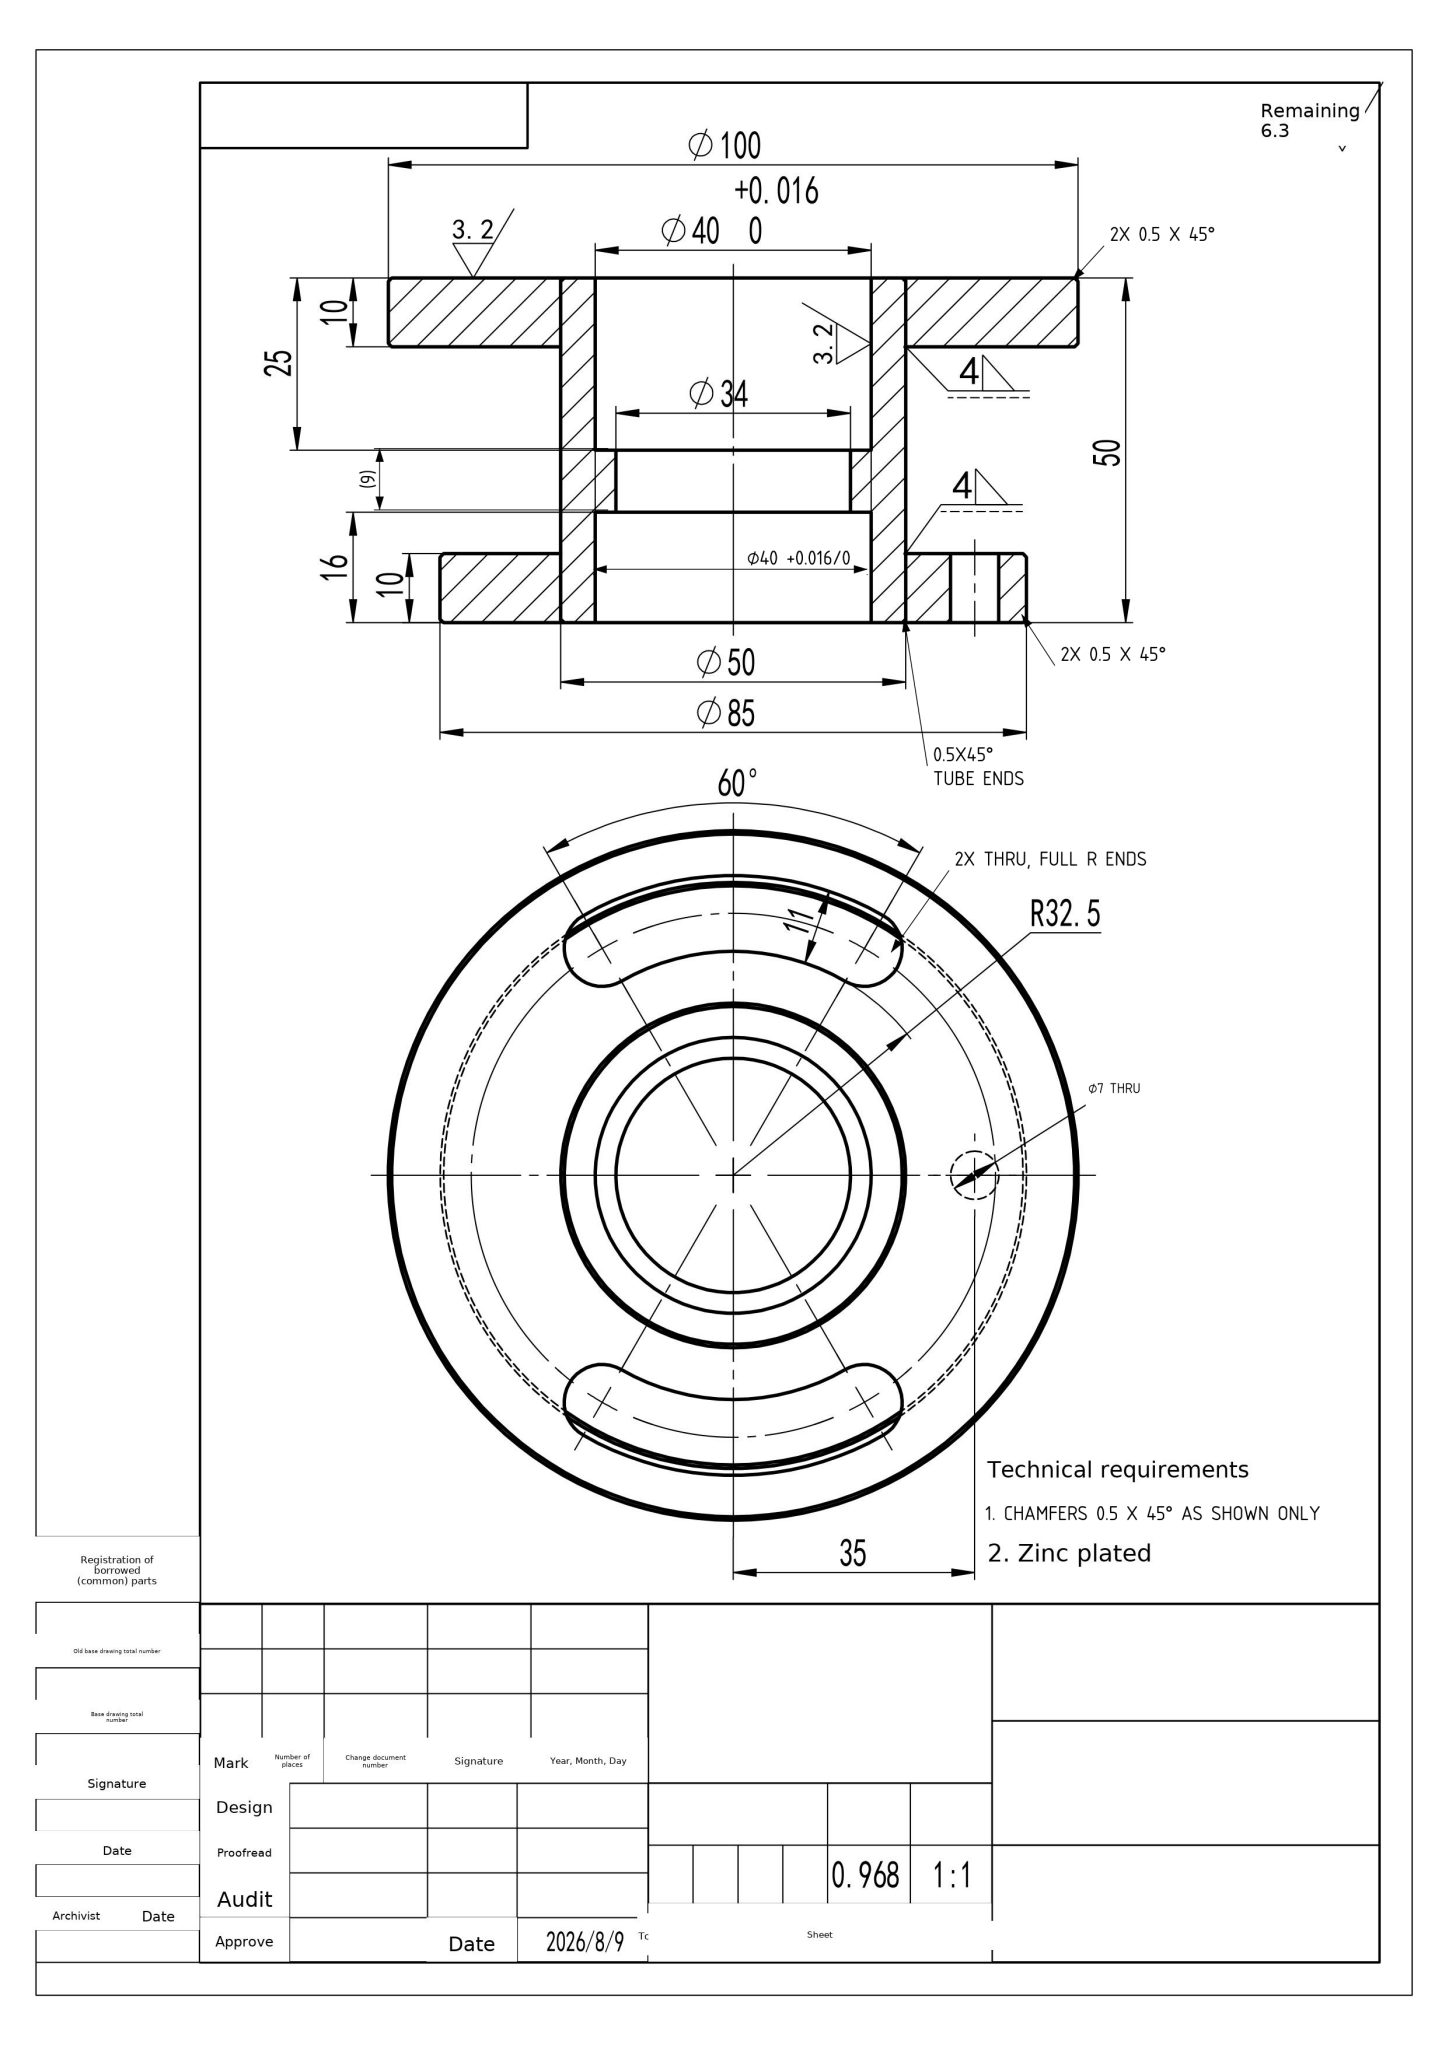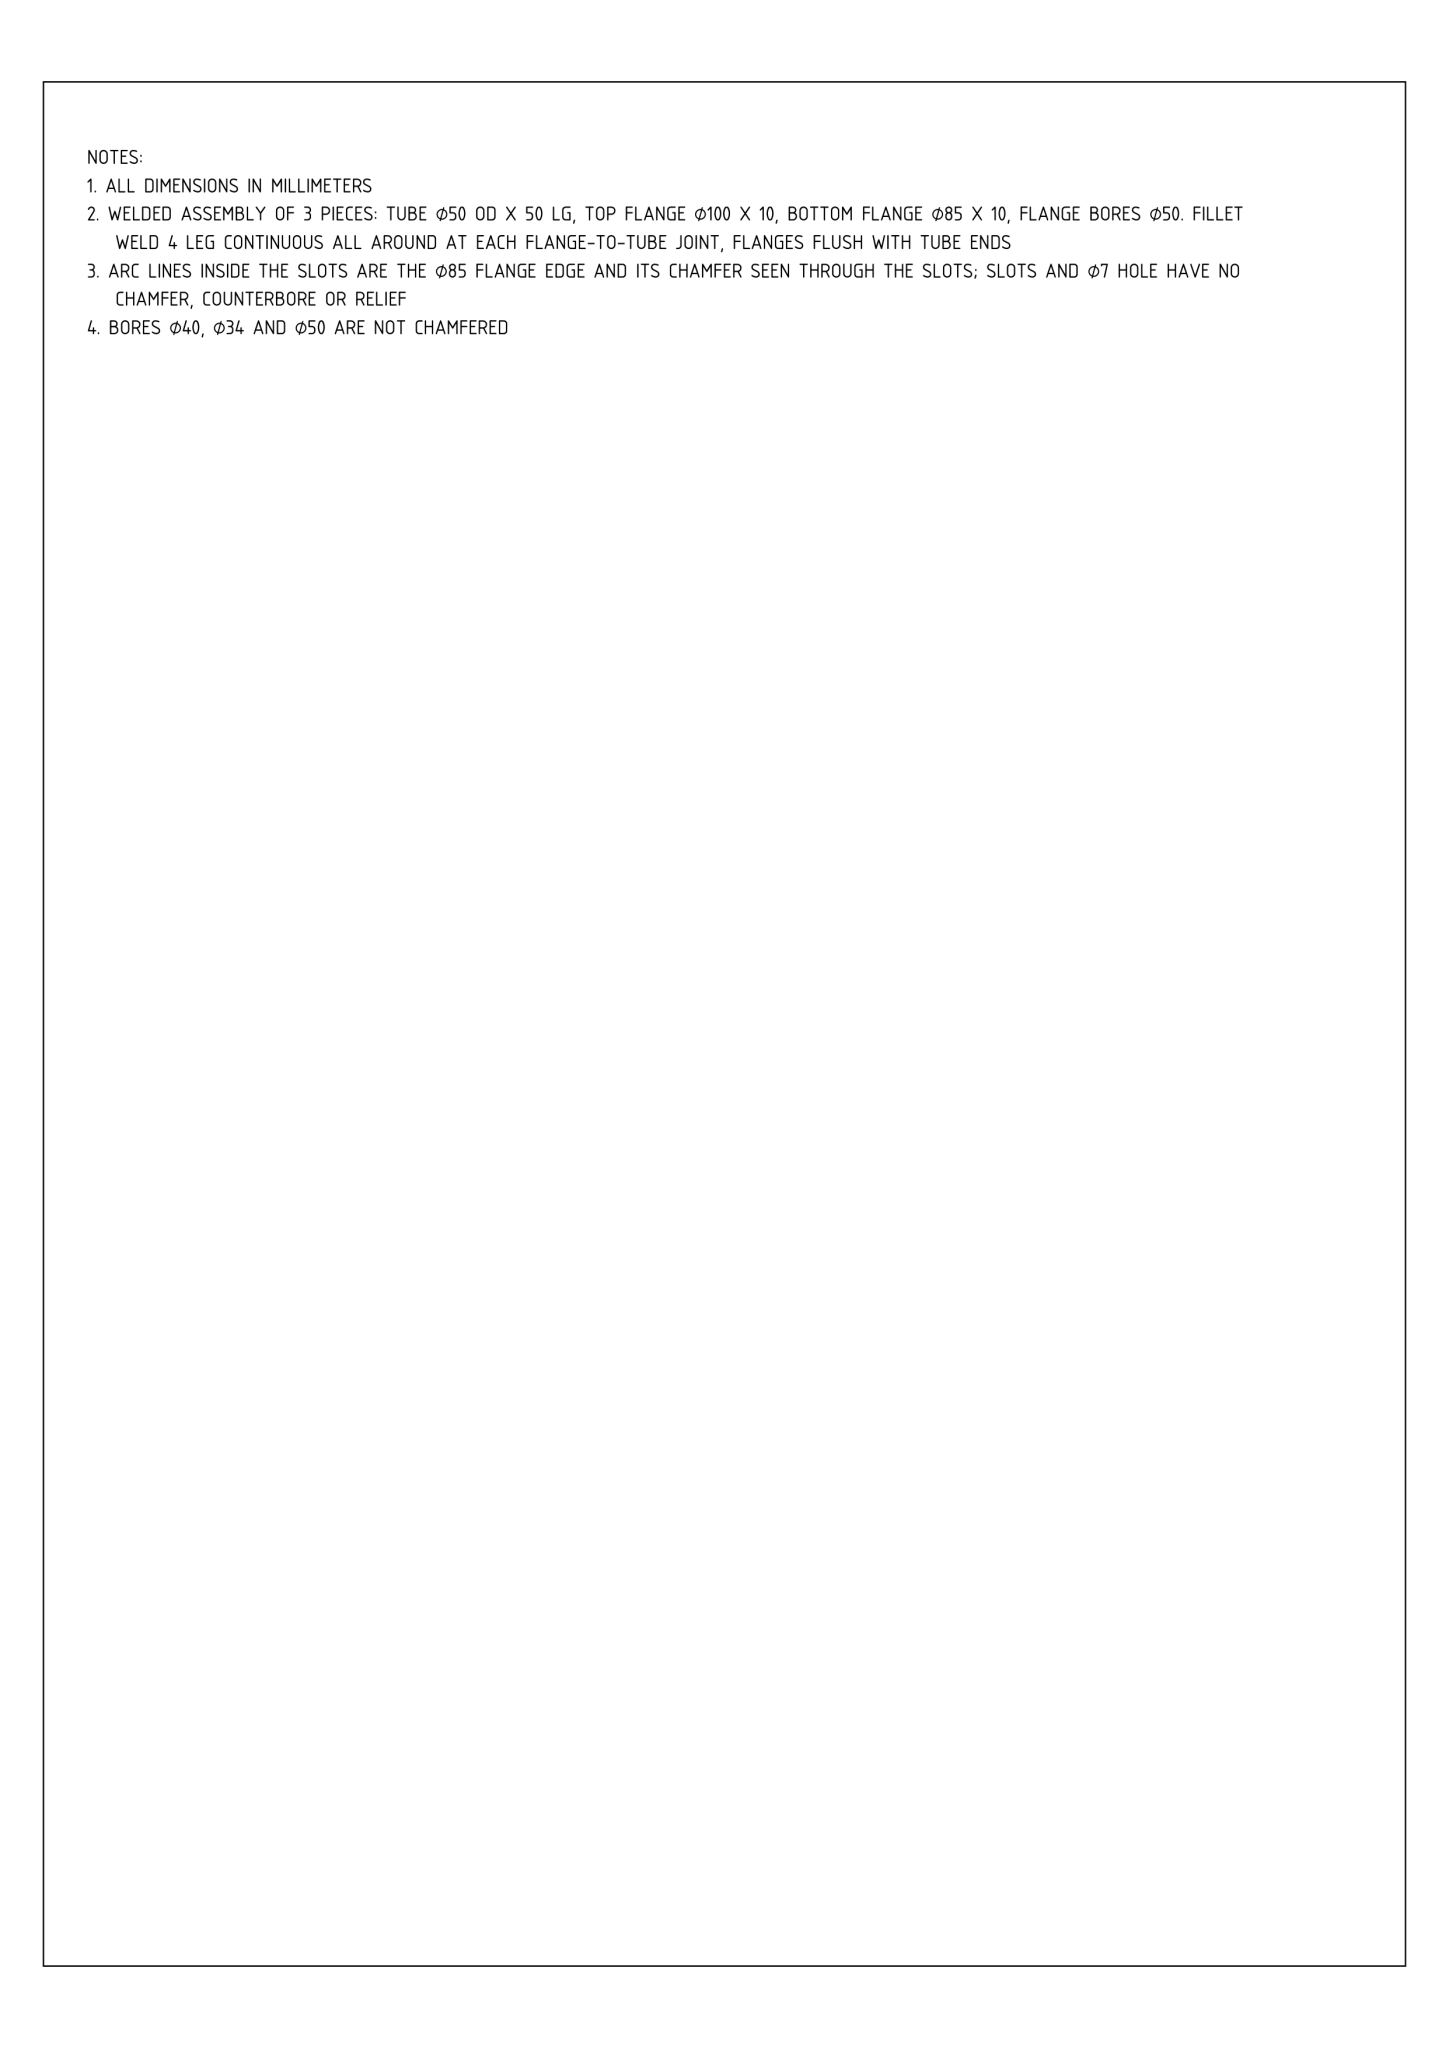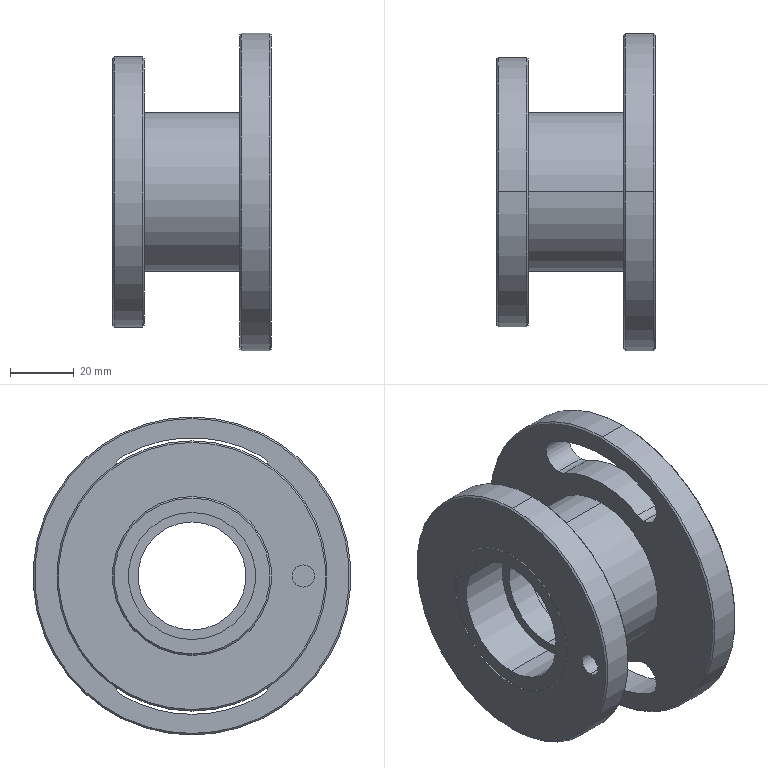Part | NX | mm | 1 solid | 50 faces | box 50 x 100 x 100 mm | volume 123272 mm3 | cylinder 30 | cone 12 | plane 8 | commonest cylinder face diameters 11 x6 50 x6 40 x4 65 x3 87 x3 7 x2 100 x2 85 x2